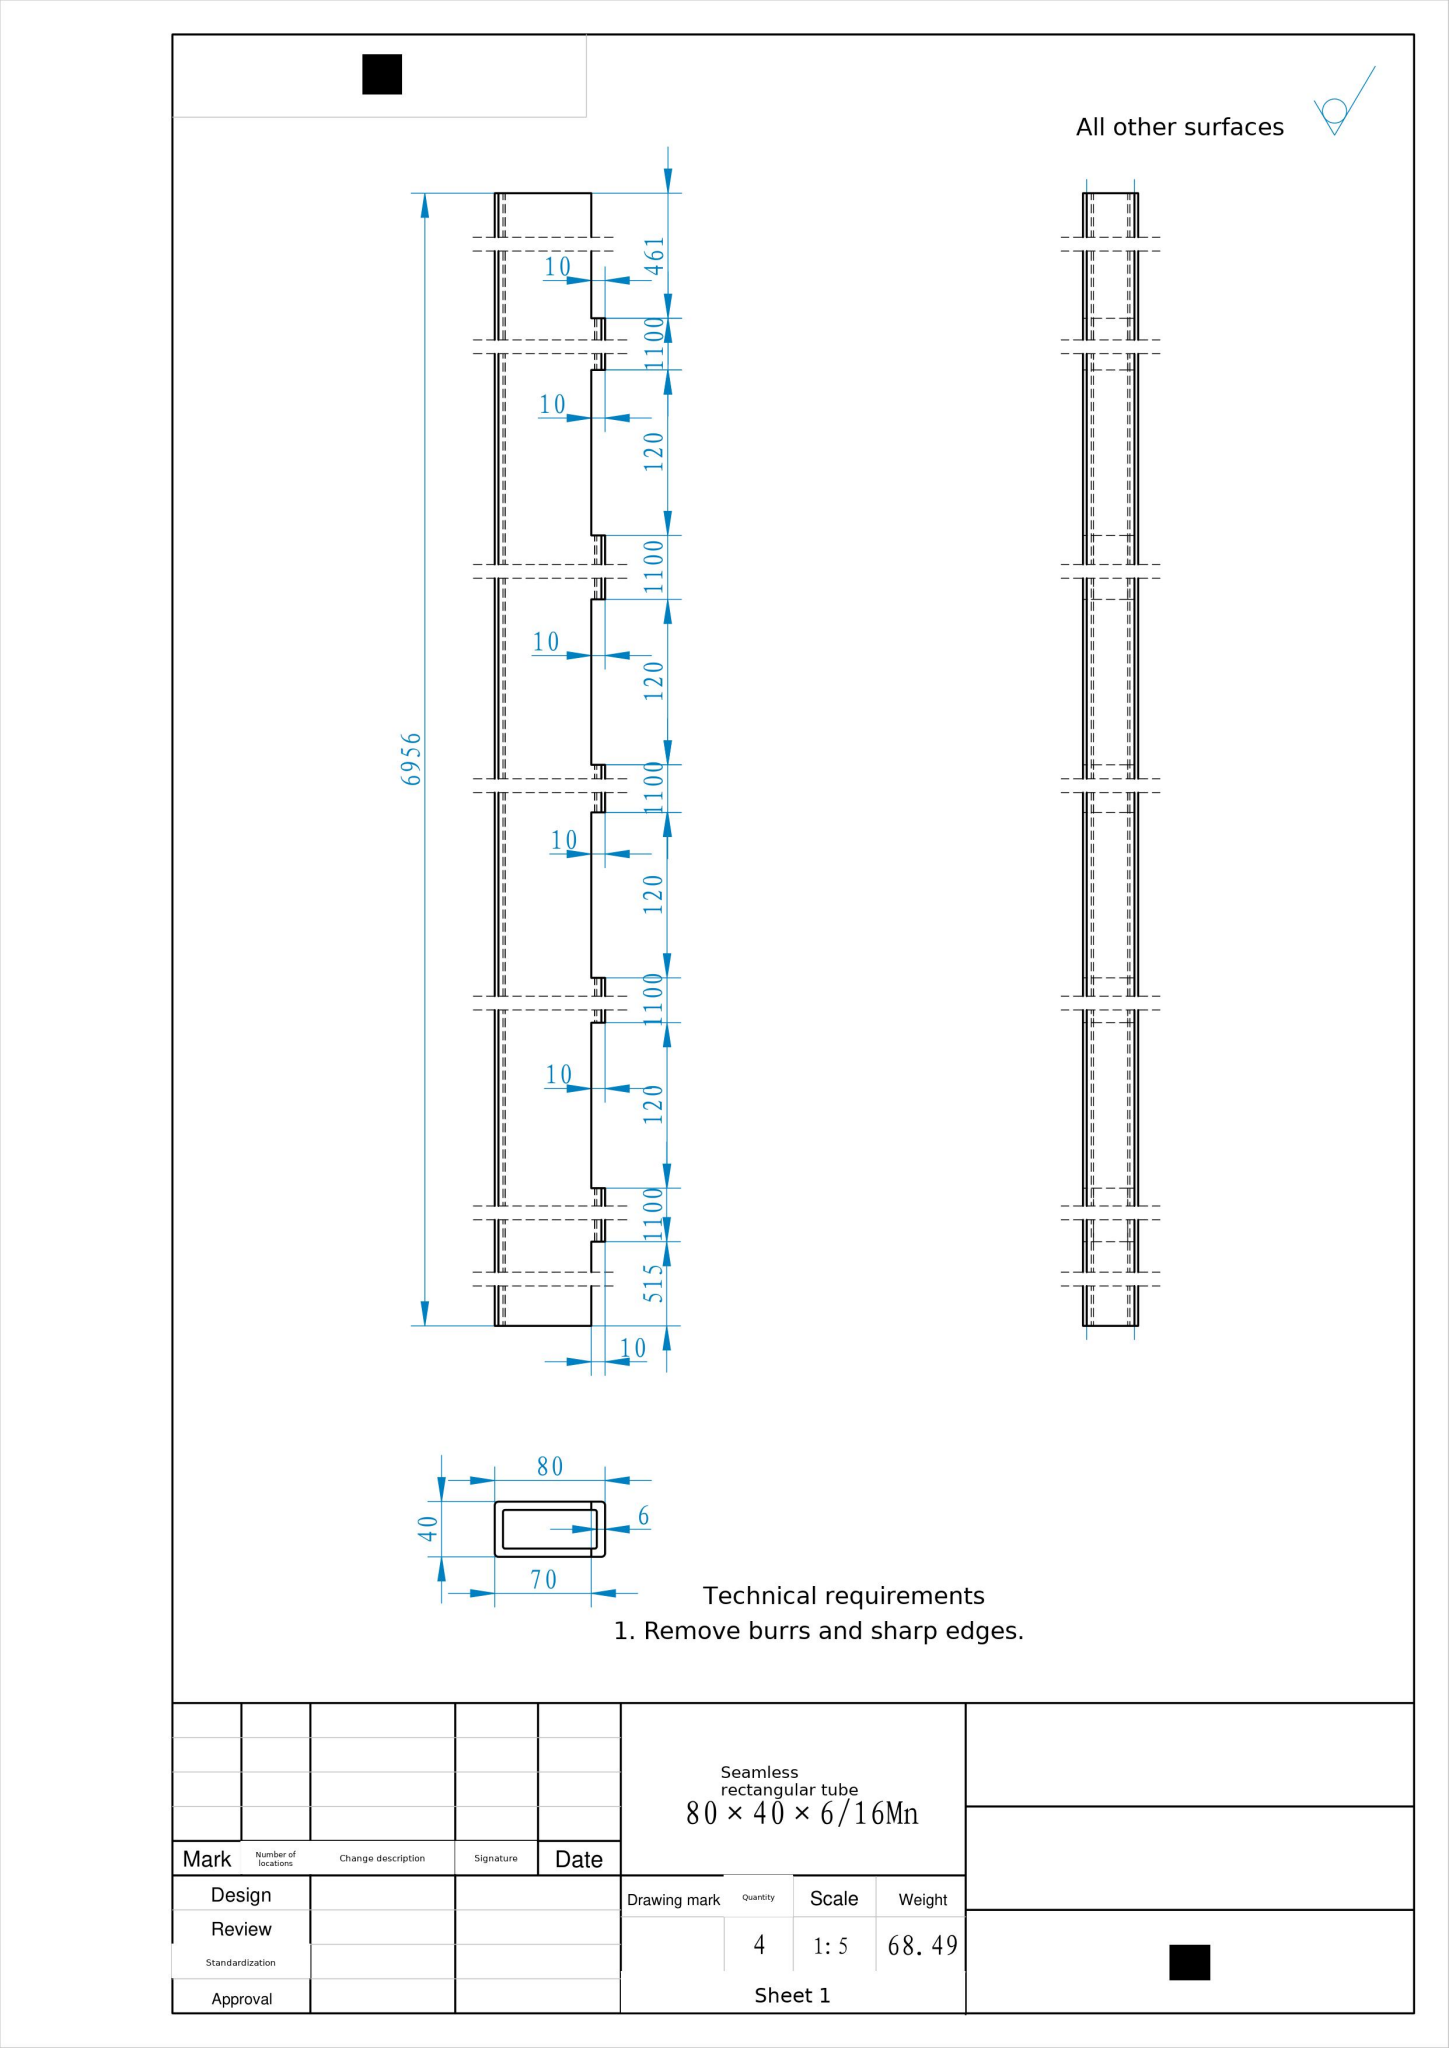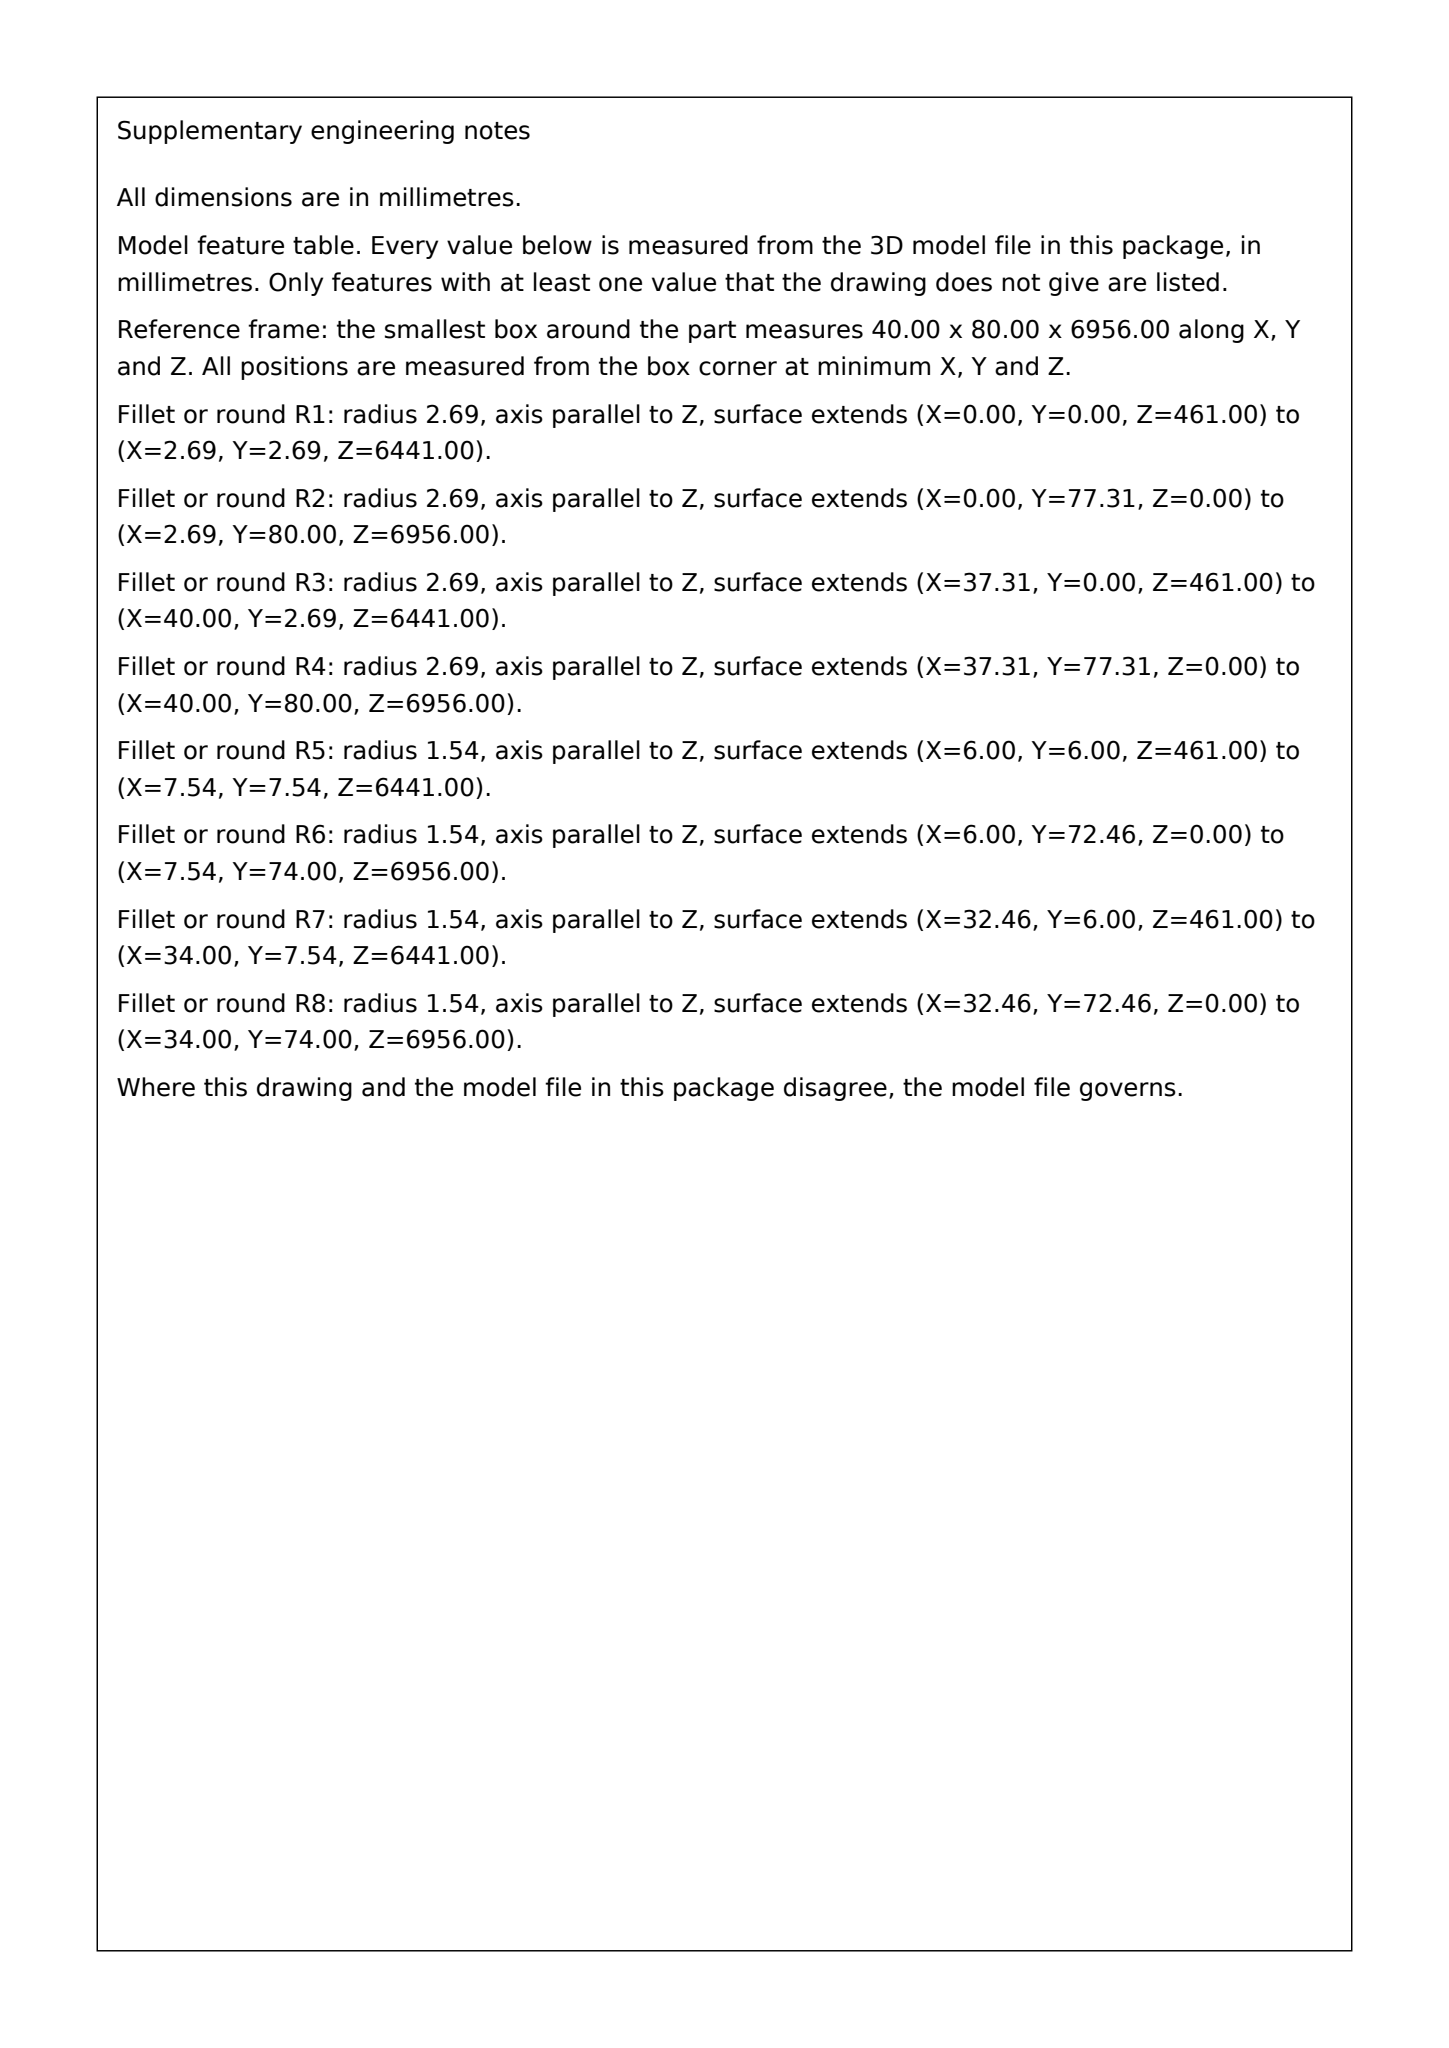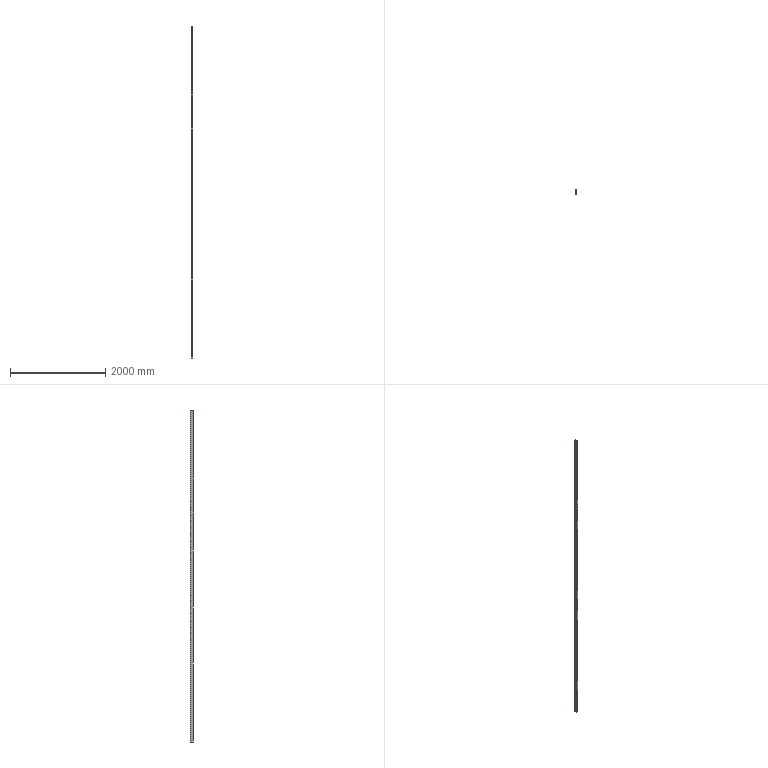Part | SolidWorks | mm | material Seamless rectangular tube 80 × 40 × 6/16Mn | 1 solid | 64 faces | box 40 x 80 x 6956 mm | volume 8569584 mm3 | plane 40 | cylinder 24 | commonest cylinder face diameters 5.384 x12 3.08 x12
build123d program:
from build123d import *

# Parameters (mm, degrees)
BOSS_EXTRUDE_DEPTH = 6956
SKETCH6_W          = 943.673
SKETCH6_H          = 101.245
SKETCH6_W_2        = 120
SKETCH6_H_2        = 61.371
SKETCH6_H_3        = 83.233
SKETCH6_W_3        = 692.094
SKETCH6_H_4        = 117.42
CUT_EXTRUDE4_DEPTH = 50


with BuildPart() as part:
    # Sketch2 → Boss-Extrude (new body)
    with BuildSketch(Plane.XY):
        with BuildLine():
            Line((-17.308, 40), (17.308, 40))
            ThreePointArc((17.308, 40), (19.212, 39.212), (20, 37.308))
            Line((20, 37.308), (20, -37.308))
            ThreePointArc((20, -37.308), (19.212, -39.212), (17.308, -40))
            Line((17.308, -40), (-17.308, -40))
            ThreePointArc((-17.308, -40), (-19.212, -39.212), (-20, -37.308))
            Line((-20, -37.308), (-20, 37.308))
            ThreePointArc((-20, 37.308), (-19.212, 39.212), (-17.308, 40))
        make_face()
        with BuildLine():
            Line((-12.46, 34), (12.46, 34))
            ThreePointArc((12.46, 34), (13.549, 33.549), (14, 32.46))
            Line((14, 32.46), (14, -32.46))
            ThreePointArc((14, -32.46), (13.549, -33.549), (12.46, -34))
            Line((12.46, -34), (-12.46, -34))
            ThreePointArc((-12.46, -34), (-13.549, -33.549), (-14, -32.46))
            Line((-14, -32.46), (-14, 32.46))
            ThreePointArc((-14, 32.46), (-13.549, 33.549), (-12.46, 34))
        make_face(mode=Mode.SUBTRACT)
    extrude(amount=BOSS_EXTRUDE_DEPTH)

    # Sketch6 → Cut-Extrude4 (cut, symmetric)
    with BuildSketch(Plane(origin=(0, 0, 0), x_dir=(0, 0, -1), z_dir=(1, 0, 0))):
        with Locations((-6912.837, -80.623)):
            Rectangle(SKETCH6_W, SKETCH6_H)
        with Locations((-5281, -60.685)):
            Rectangle(SKETCH6_W_2, SKETCH6_H_2)
        with Locations((-4061, -80.623)):
            Rectangle(SKETCH6_W_2, SKETCH6_H)
        with Locations((-2841, -80.623)):
            Rectangle(SKETCH6_W_2, SKETCH6_H)
        with Locations((-1621, -71.616)):
            Rectangle(SKETCH6_W_2, SKETCH6_H_3)
        with Locations((-114.953, -88.71)):
            Rectangle(SKETCH6_W_3, SKETCH6_H_4)
    extrude(amount=CUT_EXTRUDE4_DEPTH, both=True, mode=Mode.SUBTRACT)


solid = part.part